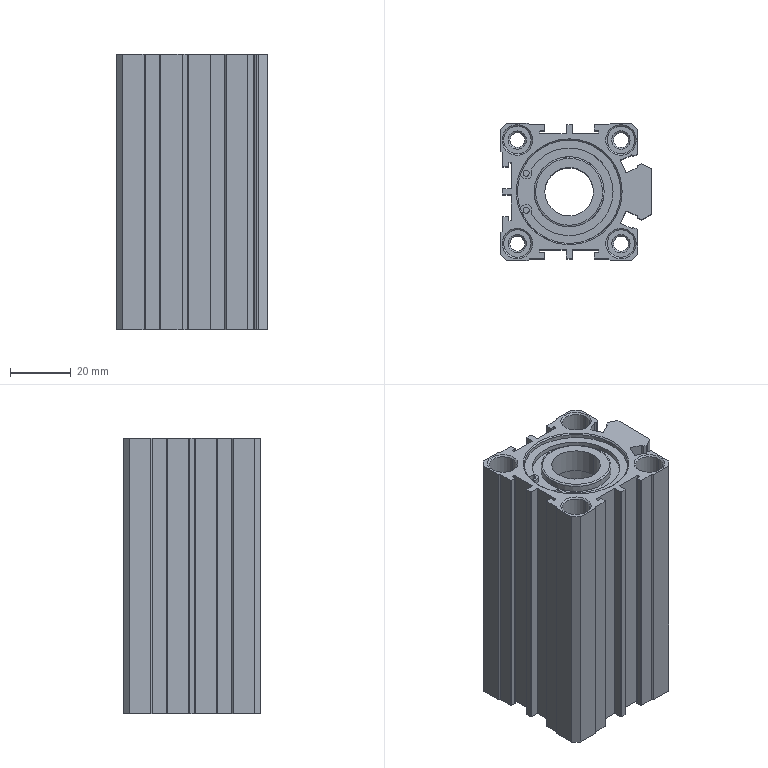Component | SolidWorks | JDAD32x50-20-SE2-1_BEN-1 | 1 solid | 289 faces | volume 94561 mm3 | cylinder 127 | plane 102 | cone 56 | spline 4 | commonest cylinder face diameters 0.4 x36 9 x16 4.917 x16 2 x12 5.2 x8 0.8 x8 3.8 x6 16 x4